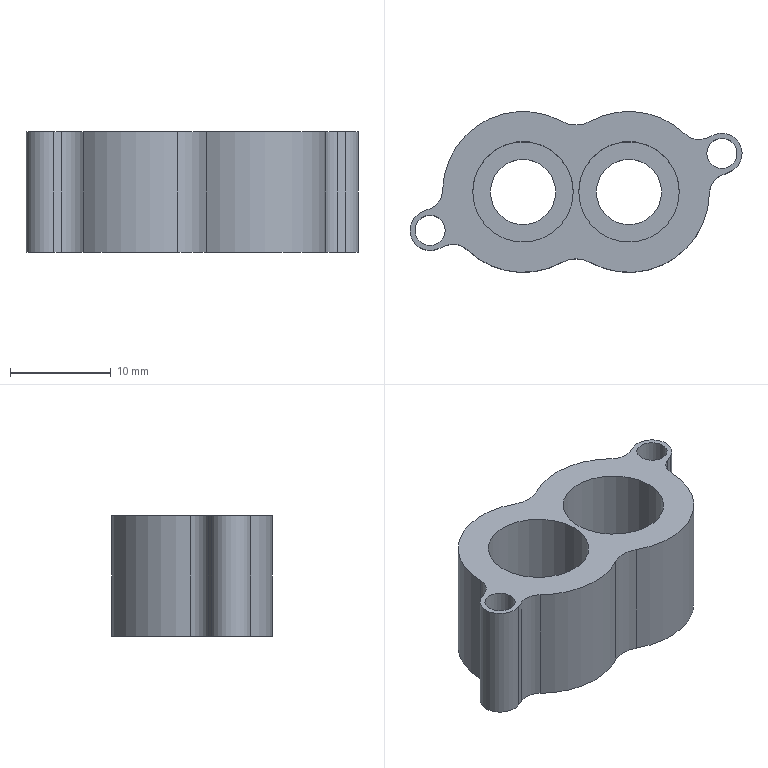Component | NX | GEAR_ROTOR_COVER | 1 solid | 26 faces | volume 2787 mm3 | cylinder 18 | plane 8 | commonest cylinder face diameters 4 x6 16 x4 6 x2 3 x2 10 x2 6.5 x2